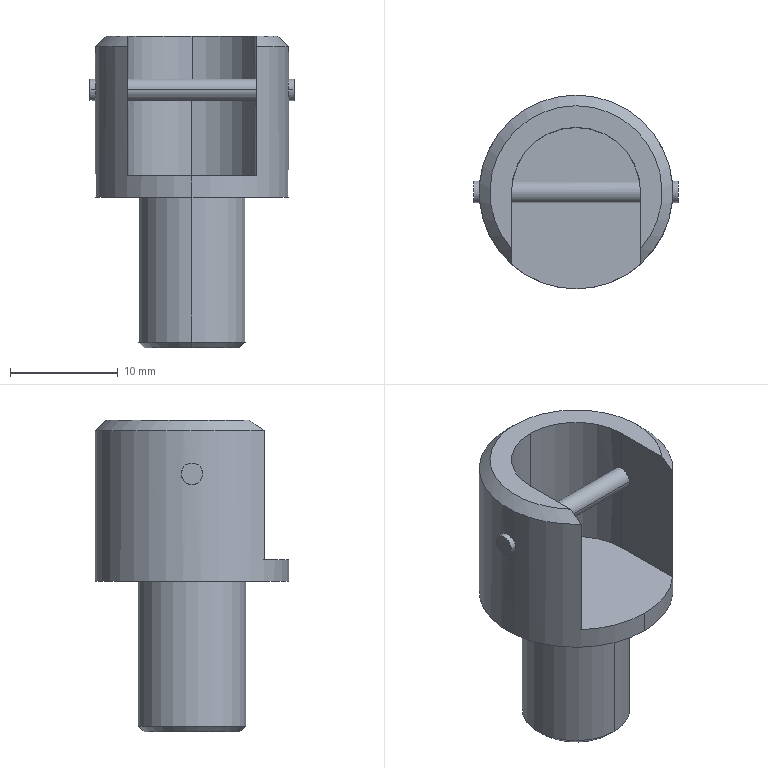Component | SolidWorks | ControlAssembly-1_UWAFN120-1_1_1-1 | 1 solid | 26 faces | box 19 x 18 x 29 mm | volume 2693 mm3 | cylinder 14 | plane 9 | cone 3 | commonest cylinder face diameters 2 x6 5.2 x2 18 x2 10 x2 12 x2
STEP:
#1=CARTESIAN_POINT('',(24.624,0.9121,20.53));
#2=VERTEX_POINT('',#1);
#3=CARTESIAN_POINT('',(24.624,0.7073,20.53));
#4=VERTEX_POINT('',#3);
#5=CARTESIAN_POINT('',(24.624,0.8097,20.53));
#6=DIRECTION('',(-0.00009864,0.,-1.));
#7=DIRECTION('',(0.,-1.,0.));
#8=AXIS2_PLACEMENT_3D('',#5,#6,#7);
#9=CIRCLE('',#8,0.1024);
#10=EDGE_CURVE('',#2,#4,#9,.T.);
#11=ORIENTED_EDGE('',*,*,#10,.F.);
#12=CARTESIAN_POINT('',(24.624,0.9121,20.136));
#13=VERTEX_POINT('',#12);
#14=CARTESIAN_POINT('',(24.624,0.9121,20.53));
#15=DIRECTION('',(-0.00009864,0.,-1.));
#16=VECTOR('',#15,39.37);
#17=LINE('',#14,#16);
#18=EDGE_CURVE('',#2,#13,#17,.T.);
#19=ORIENTED_EDGE('',*,*,#18,.T.);
#20=CARTESIAN_POINT('',(24.624,0.7073,20.136));
#21=VERTEX_POINT('',#20);
#22=CARTESIAN_POINT('',(24.624,0.8097,20.136));
#23=DIRECTION('',(-0.00009864,0.,-1.));
#24=DIRECTION('',(0.,-1.,0.));
#25=AXIS2_PLACEMENT_3D('',#22,#23,#24);
#26=CIRCLE('',#25,0.1024);
#27=EDGE_CURVE('',#13,#21,#26,.T.);
#28=ORIENTED_EDGE('',*,*,#27,.T.);
#29=CARTESIAN_POINT('',(24.624,0.7073,20.53));
#30=DIRECTION('',(-0.00009864,0.,-1.));
#31=VECTOR('',#30,39.37);
#32=LINE('',#29,#31);
#33=EDGE_CURVE('',#4,#21,#32,.T.);
#34=ORIENTED_EDGE('',*,*,#33,.F.);
#35=EDGE_LOOP('',(#11,#19,#28,#34));
#36=FACE_OUTER_BOUND('',#35,.T.);
#37=CARTESIAN_POINT('',(24.624,0.8097,20.53));
#38=DIRECTION('',(-0.00009864,0.,-1.));
#39=DIRECTION('',(0.,-1.,0.));
#40=AXIS2_PLACEMENT_3D('',#37,#38,#39);
#41=CYLINDRICAL_SURFACE('',#40,0.1024);
#42=ADVANCED_FACE('',(#36),#41,.F.);
#43=CARTESIAN_POINT('',(24.272,0.7703,21.081));
#44=VERTEX_POINT('',#43);
#45=CARTESIAN_POINT('',(24.272,0.8491,21.081));
#46=VERTEX_POINT('',#45);
#47=CARTESIAN_POINT('',(24.272,0.7703,21.081));
#48=CARTESIAN_POINT('',(24.272,0.7703,21.076));
#49=CARTESIAN_POINT('',(24.272,0.7714,21.07));
#50=CARTESIAN_POINT('',(24.272,0.7753,21.061));
#51=CARTESIAN_POINT('',(24.271,0.7782,21.057));
#52=CARTESIAN_POINT('',(24.271,0.7855,21.049));
#53=CARTESIAN_POINT('',(24.271,0.7899,21.046));
#54=CARTESIAN_POINT('',(24.27,0.7994,21.042));
#55=CARTESIAN_POINT('',(24.27,0.8045,21.041));
#56=CARTESIAN_POINT('',(24.27,0.8149,21.041));
#57=CARTESIAN_POINT('',(24.27,0.82,21.042));
#58=CARTESIAN_POINT('',(24.271,0.8295,21.046));
#59=CARTESIAN_POINT('',(24.271,0.8339,21.049));
#60=CARTESIAN_POINT('',(24.272,0.8448,21.06));
#61=CARTESIAN_POINT('',(24.272,0.8491,21.07));
#62=CARTESIAN_POINT('',(24.272,0.8491,21.081));
#63=B_SPLINE_CURVE_WITH_KNOTS('',3,(#47,#48,#49,#50,#51,#52,#53,#54,#55,#56,#57,#58,#59,#60,#61,#62),.UNSPECIFIED.,.F.,.F.,(4,2,2,2,2,2,2,4),(0.004692,0.005082,0.005473,0.005864,0.006255,0.006646,0.007037,0.007818),.UNSPECIFIED.);
#64=EDGE_CURVE('',#44,#46,#63,.T.);
#65=ORIENTED_EDGE('',*,*,#64,.T.);
#66=CARTESIAN_POINT('',(24.272,0.8491,21.081));
#67=CARTESIAN_POINT('',(24.272,0.8491,21.086));
#68=CARTESIAN_POINT('',(24.272,0.848,21.091));
#69=CARTESIAN_POINT('',(24.272,0.8441,21.101));
#70=CARTESIAN_POINT('',(24.271,0.8412,21.105));
#71=CARTESIAN_POINT('',(24.271,0.8303,21.116));
#72=CARTESIAN_POINT('',(24.27,0.8201,21.12));
#73=CARTESIAN_POINT('',(24.27,0.8045,21.12));
#74=CARTESIAN_POINT('',(24.27,0.7994,21.119));
#75=CARTESIAN_POINT('',(24.271,0.7898,21.115));
#76=CARTESIAN_POINT('',(24.271,0.7855,21.112));
#77=CARTESIAN_POINT('',(24.271,0.7782,21.105));
#78=CARTESIAN_POINT('',(24.272,0.7753,21.101));
#79=CARTESIAN_POINT('',(24.272,0.7714,21.091));
#80=CARTESIAN_POINT('',(24.272,0.7703,21.086));
#81=CARTESIAN_POINT('',(24.272,0.7703,21.081));
#82=B_SPLINE_CURVE_WITH_KNOTS('',3,(#66,#67,#68,#69,#70,#71,#72,#73,#74,#75,#76,#77,#78,#79,#80,#81),.UNSPECIFIED.,.F.,.F.,(4,2,2,2,2,2,2,4),(0.001563,0.001954,0.002345,0.003127,0.003518,0.00391,0.004301,0.004692),.UNSPECIFIED.);
#83=EDGE_CURVE('',#46,#44,#82,.T.);
#84=ORIENTED_EDGE('',*,*,#83,.T.);
#85=EDGE_LOOP('',(#65,#84));
#86=FACE_BOUND('',#85,.T.);
#87=CARTESIAN_POINT('',(24.388,0.5456,21.238));
#88=VERTEX_POINT('',#87);
#89=CARTESIAN_POINT('',(24.624,1.164,21.238));
#90=VERTEX_POINT('',#89);
#91=CARTESIAN_POINT('',(24.624,0.8097,21.238));
#92=DIRECTION('',(-0.00009864,0.,-1.));
#93=DIRECTION('',(0.,-1.,0.));
#94=AXIS2_PLACEMENT_3D('',#91,#92,#93);
#95=CIRCLE('',#94,0.3543);
#96=EDGE_CURVE('',#88,#90,#95,.T.);
#97=ORIENTED_EDGE('',*,*,#96,.T.);
#98=CARTESIAN_POINT('',(24.624,1.164,20.687));
#99=VERTEX_POINT('',#98);
#100=CARTESIAN_POINT('',(24.624,1.164,20.963));
#101=DIRECTION('',(-0.00009864,0.,-1.));
#102=VECTOR('',#101,39.37);
#103=LINE('',#100,#102);
#104=EDGE_CURVE('',#90,#99,#103,.T.);
#105=ORIENTED_EDGE('',*,*,#104,.T.);
#106=CARTESIAN_POINT('',(24.624,0.4554,20.687));
#107=VERTEX_POINT('',#106);
#108=CARTESIAN_POINT('',(24.624,0.8097,20.687));
#109=DIRECTION('',(0.00009864,-0.,1.));
#110=DIRECTION('',(0.,-1.,0.));
#111=AXIS2_PLACEMENT_3D('',#108,#109,#110);
#112=CIRCLE('',#111,0.3543);
#113=EDGE_CURVE('',#99,#107,#112,.T.);
#114=ORIENTED_EDGE('',*,*,#113,.T.);
#115=CARTESIAN_POINT('',(24.624,0.4554,20.766));
#116=VERTEX_POINT('',#115);
#117=CARTESIAN_POINT('',(24.624,0.4554,20.963));
#118=DIRECTION('',(-0.00009864,0.,-1.));
#119=VECTOR('',#118,39.37);
#120=LINE('',#117,#119);
#121=EDGE_CURVE('',#116,#107,#120,.T.);
#122=ORIENTED_EDGE('',*,*,#121,.F.);
#123=CARTESIAN_POINT('',(24.388,0.5456,20.766));
#124=VERTEX_POINT('',#123);
#125=CARTESIAN_POINT('',(24.624,0.8097,20.766));
#126=DIRECTION('',(-0.00009864,0.,-1.));
#127=DIRECTION('',(0.,-1.,0.));
#128=AXIS2_PLACEMENT_3D('',#125,#126,#127);
#129=CIRCLE('',#128,0.3543);
#130=EDGE_CURVE('',#116,#124,#129,.T.);
#131=ORIENTED_EDGE('',*,*,#130,.T.);
#132=CARTESIAN_POINT('',(24.388,0.5456,20.963));
#133=DIRECTION('',(0.00009864,-0.,1.));
#134=VECTOR('',#133,39.37);
#135=LINE('',#132,#134);
#136=EDGE_CURVE('',#124,#88,#135,.T.);
#137=ORIENTED_EDGE('',*,*,#136,.T.);
#138=EDGE_LOOP('',(#97,#105,#114,#122,#131,#137));
#139=FACE_OUTER_BOUND('',#138,.T.);
#140=CARTESIAN_POINT('',(24.624,0.8097,20.963));
#141=DIRECTION('',(-0.00009864,0.,-1.));
#142=DIRECTION('',(0.,-1.,0.));
#143=AXIS2_PLACEMENT_3D('',#140,#141,#142);
#144=CYLINDRICAL_SURFACE('',#143,0.3543);
#145=ADVANCED_FACE('',(#86,#139),#144,.T.);
#146=CARTESIAN_POINT('',(24.998,0.7703,21.081));
#147=VERTEX_POINT('',#146);
#148=CARTESIAN_POINT('',(24.998,0.8491,21.081));
#149=VERTEX_POINT('',#148);
#150=CARTESIAN_POINT('',(24.998,0.8097,21.081));
#151=DIRECTION('',(-1.,-0.,0.00009864));
#152=DIRECTION('',(0.,-1.,0.));
#153=AXIS2_PLACEMENT_3D('',#150,#151,#152);
#154=CIRCLE('',#153,0.03937);
#155=EDGE_CURVE('',#147,#149,#154,.T.);
#156=ORIENTED_EDGE('',*,*,#155,.T.);
#157=CARTESIAN_POINT('',(24.976,0.8491,21.081));
#158=VERTEX_POINT('',#157);
#159=CARTESIAN_POINT('',(24.624,0.8491,21.081));
#160=DIRECTION('',(-1.,-0.,0.00009864));
#161=VECTOR('',#160,39.37);
#162=LINE('',#159,#161);
#163=EDGE_CURVE('',#149,#158,#162,.T.);
#164=ORIENTED_EDGE('',*,*,#163,.T.);
#165=CARTESIAN_POINT('',(24.976,0.7703,21.081));
#166=VERTEX_POINT('',#165);
#167=CARTESIAN_POINT('',(24.976,0.7703,21.081));
#168=CARTESIAN_POINT('',(24.976,0.7703,21.086));
#169=CARTESIAN_POINT('',(24.977,0.7714,21.091));
#170=CARTESIAN_POINT('',(24.977,0.7753,21.1));
#171=CARTESIAN_POINT('',(24.977,0.7782,21.105));
#172=CARTESIAN_POINT('',(24.978,0.7855,21.112));
#173=CARTESIAN_POINT('',(24.978,0.7899,21.115));
#174=CARTESIAN_POINT('',(24.979,0.7994,21.119));
#175=CARTESIAN_POINT('',(24.979,0.8045,21.12));
#176=CARTESIAN_POINT('',(24.979,0.8149,21.12));
#177=CARTESIAN_POINT('',(24.979,0.82,21.119));
#178=CARTESIAN_POINT('',(24.978,0.8295,21.115));
#179=CARTESIAN_POINT('',(24.978,0.8339,21.112));
#180=CARTESIAN_POINT('',(24.977,0.8448,21.101));
#181=CARTESIAN_POINT('',(24.976,0.8491,21.091));
#182=CARTESIAN_POINT('',(24.976,0.8491,21.081));
#183=B_SPLINE_CURVE_WITH_KNOTS('',3,(#167,#168,#169,#170,#171,#172,#173,#174,#175,#176,#177,#178,#179,#180,#181,#182),.UNSPECIFIED.,.F.,.F.,(4,2,2,2,2,2,2,4),(0.004692,0.005082,0.005473,0.005864,0.006255,0.006646,0.007037,0.007818),.UNSPECIFIED.);
#184=EDGE_CURVE('',#166,#158,#183,.T.);
#185=ORIENTED_EDGE('',*,*,#184,.F.);
#186=CARTESIAN_POINT('',(24.624,0.7703,21.081));
#187=DIRECTION('',(-1.,-0.,0.00009864));
#188=VECTOR('',#187,39.37);
#189=LINE('',#186,#188);
#190=EDGE_CURVE('',#147,#166,#189,.T.);
#191=ORIENTED_EDGE('',*,*,#190,.F.);
#192=EDGE_LOOP('',(#156,#164,#185,#191));
#193=FACE_OUTER_BOUND('',#192,.T.);
#194=CARTESIAN_POINT('',(24.624,0.8097,21.081));
#195=DIRECTION('',(-1.,-0.,0.00009864));
#196=DIRECTION('',(0.,-1.,0.));
#197=AXIS2_PLACEMENT_3D('',#194,#195,#196);
#198=CYLINDRICAL_SURFACE('',#197,0.03937);
#199=ADVANCED_FACE('',(#193),#198,.T.);
#200=ORIENTED_EDGE('',*,*,#83,.F.);
#201=CARTESIAN_POINT('',(24.25,0.8491,21.081));
#202=VERTEX_POINT('',#201);
#203=CARTESIAN_POINT('',(24.624,0.8491,21.081));
#204=DIRECTION('',(-1.,-0.,0.00009864));
#205=VECTOR('',#204,39.37);
#206=LINE('',#203,#205);
#207=EDGE_CURVE('',#46,#202,#206,.T.);
#208=ORIENTED_EDGE('',*,*,#207,.T.);
#209=CARTESIAN_POINT('',(24.25,0.7703,21.081));
#210=VERTEX_POINT('',#209);
#211=CARTESIAN_POINT('',(24.25,0.8097,21.081));
#212=DIRECTION('',(1.,0.,-0.00009864));
#213=DIRECTION('',(0.,-1.,-0.));
#214=AXIS2_PLACEMENT_3D('',#211,#212,#213);
#215=CIRCLE('',#214,0.03937);
#216=EDGE_CURVE('',#202,#210,#215,.T.);
#217=ORIENTED_EDGE('',*,*,#216,.T.);
#218=CARTESIAN_POINT('',(24.624,0.7703,21.081));
#219=DIRECTION('',(-1.,-0.,0.00009864));
#220=VECTOR('',#219,39.37);
#221=LINE('',#218,#220);
#222=EDGE_CURVE('',#44,#210,#221,.T.);
#223=ORIENTED_EDGE('',*,*,#222,.F.);
#224=EDGE_LOOP('',(#200,#208,#217,#223));
#225=FACE_OUTER_BOUND('',#224,.T.);
#226=CARTESIAN_POINT('',(24.624,0.8097,21.081));
#227=DIRECTION('',(-1.,-0.,0.00009864));
#228=DIRECTION('',(0.,-1.,0.));
#229=AXIS2_PLACEMENT_3D('',#226,#227,#228);
#230=CYLINDRICAL_SURFACE('',#229,0.03937);
#231=ADVANCED_FACE('',(#225),#230,.T.);
#232=CARTESIAN_POINT('',(24.624,1.007,20.687));
#233=VERTEX_POINT('',#232);
#234=CARTESIAN_POINT('',(24.624,0.6129,20.687));
#235=VERTEX_POINT('',#234);
#236=CARTESIAN_POINT('',(24.624,0.8097,20.687));
#237=DIRECTION('',(0.00009864,-0.,1.));
#238=DIRECTION('',(0.,-1.,0.));
#239=AXIS2_PLACEMENT_3D('',#236,#237,#238);
#240=CIRCLE('',#239,0.1969);
#241=EDGE_CURVE('',#233,#235,#240,.T.);
#242=ORIENTED_EDGE('',*,*,#241,.F.);
#243=CARTESIAN_POINT('',(24.624,1.007,20.157));
#244=VERTEX_POINT('',#243);
#245=CARTESIAN_POINT('',(24.624,1.007,20.422));
#246=DIRECTION('',(-0.00009864,0.,-1.));
#247=VECTOR('',#246,39.37);
#248=LINE('',#245,#247);
#249=EDGE_CURVE('',#233,#244,#248,.T.);
#250=ORIENTED_EDGE('',*,*,#249,.T.);
#251=CARTESIAN_POINT('',(24.624,0.6129,20.157));
#252=VERTEX_POINT('',#251);
#253=CARTESIAN_POINT('',(24.624,0.8097,20.157));
#254=DIRECTION('',(0.00009864,-0.,1.));
#255=DIRECTION('',(0.,-1.,0.));
#256=AXIS2_PLACEMENT_3D('',#253,#254,#255);
#257=CIRCLE('',#256,0.1969);
#258=EDGE_CURVE('',#244,#252,#257,.T.);
#259=ORIENTED_EDGE('',*,*,#258,.T.);
#260=CARTESIAN_POINT('',(24.624,0.6129,20.422));
#261=DIRECTION('',(-0.00009864,0.,-1.));
#262=VECTOR('',#261,39.37);
#263=LINE('',#260,#262);
#264=EDGE_CURVE('',#235,#252,#263,.T.);
#265=ORIENTED_EDGE('',*,*,#264,.F.);
#266=EDGE_LOOP('',(#242,#250,#259,#265));
#267=FACE_OUTER_BOUND('',#266,.T.);
#268=CARTESIAN_POINT('',(24.624,0.8097,20.422));
#269=DIRECTION('',(-0.00009864,0.,-1.));
#270=DIRECTION('',(0.,-1.,0.));
#271=AXIS2_PLACEMENT_3D('',#268,#269,#270);
#272=CYLINDRICAL_SURFACE('',#271,0.1969);
#273=ADVANCED_FACE('',(#267),#272,.T.);
#274=CARTESIAN_POINT('',(24.624,0.9852,20.136));
#275=VERTEX_POINT('',#274);
#276=CARTESIAN_POINT('',(24.624,0.6342,20.136));
#277=VERTEX_POINT('',#276);
#278=CARTESIAN_POINT('',(24.624,0.8097,20.136));
#279=DIRECTION('',(0.00009864,0.,1.));
#280=DIRECTION('',(0.,1.,0.));
#281=AXIS2_PLACEMENT_3D('',#278,#279,#280);
#282=CIRCLE('',#281,0.1755);
#283=EDGE_CURVE('',#275,#277,#282,.T.);
#284=ORIENTED_EDGE('',*,*,#283,.T.);
#285=CARTESIAN_POINT('',(24.624,0.6129,20.157));
#286=DIRECTION('',(0.00006975,-0.7071,0.7071));
#287=VECTOR('',#286,39.37);
#288=LINE('',#285,#287);
#289=EDGE_CURVE('',#277,#252,#288,.T.);
#290=ORIENTED_EDGE('',*,*,#289,.T.);
#291=ORIENTED_EDGE('',*,*,#258,.F.);
#292=CARTESIAN_POINT('',(24.624,1.007,20.157));
#293=DIRECTION('',(0.00006975,0.7071,0.7071));
#294=VECTOR('',#293,39.37);
#295=LINE('',#292,#294);
#296=EDGE_CURVE('',#275,#244,#295,.T.);
#297=ORIENTED_EDGE('',*,*,#296,.F.);
#298=EDGE_LOOP('',(#284,#290,#291,#297));
#299=FACE_OUTER_BOUND('',#298,.T.);
#300=CARTESIAN_POINT('',(24.624,0.8097,20.157));
#301=DIRECTION('',(0.00009864,0.,1.));
#302=DIRECTION('',(0.,1.,0.));
#303=AXIS2_PLACEMENT_3D('',#300,#301,#302);
#304=CONICAL_SURFACE('',#303,0.1969,0.7854);
#305=ADVANCED_FACE('',(#299),#304,.T.);
#306=CARTESIAN_POINT('',(24.861,0.8097,21.12));
#307=VERTEX_POINT('',#306);
#308=CARTESIAN_POINT('',(24.857,0.8491,21.081));
#309=VERTEX_POINT('',#308);
#310=CARTESIAN_POINT('',(24.861,0.8097,21.12));
#311=CARTESIAN_POINT('',(24.861,0.8149,21.12));
#312=CARTESIAN_POINT('',(24.86,0.82,21.119));
#313=CARTESIAN_POINT('',(24.86,0.8296,21.115));
#314=CARTESIAN_POINT('',(24.859,0.8339,21.112));
#315=CARTESIAN_POINT('',(24.858,0.8412,21.105));
#316=CARTESIAN_POINT('',(24.858,0.8441,21.1));
#317=CARTESIAN_POINT('',(24.857,0.848,21.091));
#318=CARTESIAN_POINT('',(24.857,0.8491,21.086));
#319=CARTESIAN_POINT('',(24.857,0.8491,21.081));
#320=B_SPLINE_CURVE_WITH_KNOTS('',3,(#310,#311,#312,#313,#314,#315,#316,#317,#318,#319),.UNSPECIFIED.,.F.,.F.,(4,2,2,2,4),(0.,0.0003916,0.0007832,0.001175,0.001566),.UNSPECIFIED.);
#321=EDGE_CURVE('',#307,#309,#320,.T.);
#322=ORIENTED_EDGE('',*,*,#321,.T.);
#323=CARTESIAN_POINT('',(24.391,0.8491,21.081));
#324=VERTEX_POINT('',#323);
#325=CARTESIAN_POINT('',(24.624,0.8491,21.081));
#326=DIRECTION('',(-1.,-0.,0.00009864));
#327=VECTOR('',#326,39.37);
#328=LINE('',#325,#327);
#329=EDGE_CURVE('',#309,#324,#328,.T.);
#330=ORIENTED_EDGE('',*,*,#329,.T.);
#331=CARTESIAN_POINT('',(24.388,0.8097,21.12));
#332=VERTEX_POINT('',#331);
#333=CARTESIAN_POINT('',(24.391,0.8491,21.081));
#334=CARTESIAN_POINT('',(24.391,0.8491,21.086));
#335=CARTESIAN_POINT('',(24.391,0.848,21.091));
#336=CARTESIAN_POINT('',(24.391,0.8441,21.101));
#337=CARTESIAN_POINT('',(24.39,0.8412,21.105));
#338=CARTESIAN_POINT('',(24.389,0.8339,21.112));
#339=CARTESIAN_POINT('',(24.389,0.8296,21.115));
#340=CARTESIAN_POINT('',(24.388,0.82,21.119));
#341=CARTESIAN_POINT('',(24.388,0.8149,21.12));
#342=CARTESIAN_POINT('',(24.388,0.8097,21.12));
#343=B_SPLINE_CURVE_WITH_KNOTS('',3,(#333,#334,#335,#336,#337,#338,#339,#340,#341,#342),.UNSPECIFIED.,.F.,.F.,(4,2,2,2,4),(0.001566,0.001958,0.002349,0.00274,0.003131),.UNSPECIFIED.);
#344=EDGE_CURVE('',#324,#332,#343,.T.);
#345=ORIENTED_EDGE('',*,*,#344,.T.);
#346=CARTESIAN_POINT('',(24.388,0.7703,21.081));
#347=VERTEX_POINT('',#346);
#348=CARTESIAN_POINT('',(24.388,0.8097,21.081));
#349=DIRECTION('',(1.,0.,-0.00009864));
#350=DIRECTION('',(0.,-1.,-0.));
#351=AXIS2_PLACEMENT_3D('',#348,#349,#350);
#352=CIRCLE('',#351,0.03937);
#353=EDGE_CURVE('',#332,#347,#352,.T.);
#354=ORIENTED_EDGE('',*,*,#353,.T.);
#355=CARTESIAN_POINT('',(24.861,0.7703,21.081));
#356=VERTEX_POINT('',#355);
#357=CARTESIAN_POINT('',(24.624,0.7703,21.081));
#358=DIRECTION('',(-1.,-0.,0.00009864));
#359=VECTOR('',#358,39.37);
#360=LINE('',#357,#359);
#361=EDGE_CURVE('',#356,#347,#360,.T.);
#362=ORIENTED_EDGE('',*,*,#361,.F.);
#363=CARTESIAN_POINT('',(24.861,0.8097,21.081));
#364=DIRECTION('',(-1.,-0.,0.00009864));
#365=DIRECTION('',(0.,-1.,0.));
#366=AXIS2_PLACEMENT_3D('',#363,#364,#365);
#367=CIRCLE('',#366,0.03937);
#368=EDGE_CURVE('',#356,#307,#367,.T.);
#369=ORIENTED_EDGE('',*,*,#368,.T.);
#370=EDGE_LOOP('',(#322,#330,#345,#354,#362,#369));
#371=FACE_OUTER_BOUND('',#370,.T.);
#372=CARTESIAN_POINT('',(24.624,0.8097,21.081));
#373=DIRECTION('',(-1.,-0.,0.00009864));
#374=DIRECTION('',(0.,-1.,0.));
#375=AXIS2_PLACEMENT_3D('',#372,#373,#374);
#376=CYLINDRICAL_SURFACE('',#375,0.03937);
#377=ADVANCED_FACE('',(#371),#376,.T.);
#378=CARTESIAN_POINT('',(24.624,1.046,20.766));
#379=VERTEX_POINT('',#378);
#380=CARTESIAN_POINT('',(24.388,0.8097,20.766));
#381=VERTEX_POINT('',#380);
#382=CARTESIAN_POINT('',(24.624,0.8097,20.766));
#383=DIRECTION('',(0.00009864,-0.,1.));
#384=DIRECTION('',(0.,1.,0.));
#385=AXIS2_PLACEMENT_3D('',#382,#383,#384);
#386=CIRCLE('',#385,0.2362);
#387=EDGE_CURVE('',#379,#381,#386,.T.);
#388=ORIENTED_EDGE('',*,*,#387,.F.);
#389=CARTESIAN_POINT('',(24.624,1.046,21.278));
#390=VERTEX_POINT('',#389);
#391=CARTESIAN_POINT('',(24.624,1.046,21.278));
#392=DIRECTION('',(0.00009864,-0.,1.));
#393=VECTOR('',#392,39.37);
#394=LINE('',#391,#393);
#395=EDGE_CURVE('',#379,#390,#394,.T.);
#396=ORIENTED_EDGE('',*,*,#395,.T.);
#397=CARTESIAN_POINT('',(24.388,0.8097,21.278));
#398=VERTEX_POINT('',#397);
#399=CARTESIAN_POINT('',(24.624,0.8097,21.278));
#400=DIRECTION('',(-0.00009864,0.,-1.));
#401=DIRECTION('',(0.,1.,0.));
#402=AXIS2_PLACEMENT_3D('',#399,#400,#401);
#403=CIRCLE('',#402,0.2362);
#404=EDGE_CURVE('',#398,#390,#403,.T.);
#405=ORIENTED_EDGE('',*,*,#404,.F.);
#406=CARTESIAN_POINT('',(24.388,0.8097,21.278));
#407=DIRECTION('',(-0.00009864,0.,-1.));
#408=VECTOR('',#407,39.37);
#409=LINE('',#406,#408);
#410=EDGE_CURVE('',#398,#332,#409,.T.);
#411=ORIENTED_EDGE('',*,*,#410,.T.);
#412=ORIENTED_EDGE('',*,*,#344,.F.);
#413=CARTESIAN_POINT('',(24.388,0.8097,21.041));
#414=VERTEX_POINT('',#413);
#415=CARTESIAN_POINT('',(24.388,0.8097,21.041));
#416=CARTESIAN_POINT('',(24.388,0.8149,21.041));
#417=CARTESIAN_POINT('',(24.388,0.82,21.042));
#418=CARTESIAN_POINT('',(24.389,0.8296,21.046));
#419=CARTESIAN_POINT('',(24.389,0.8339,21.049));
#420=CARTESIAN_POINT('',(24.39,0.8412,21.057));
#421=CARTESIAN_POINT('',(24.391,0.8441,21.061));
#422=CARTESIAN_POINT('',(24.391,0.848,21.07));
#423=CARTESIAN_POINT('',(24.391,0.8491,21.076));
#424=CARTESIAN_POINT('',(24.391,0.8491,21.081));
#425=B_SPLINE_CURVE_WITH_KNOTS('',3,(#415,#416,#417,#418,#419,#420,#421,#422,#423,#424),.UNSPECIFIED.,.F.,.F.,(4,2,2,2,4),(0.,0.0003916,0.0007832,0.001175,0.001566),.UNSPECIFIED.);
#426=EDGE_CURVE('',#414,#324,#425,.T.);
#427=ORIENTED_EDGE('',*,*,#426,.F.);
#428=CARTESIAN_POINT('',(24.388,0.8097,21.278));
#429=DIRECTION('',(-0.00009864,0.,-1.));
#430=VECTOR('',#429,39.37);
#431=LINE('',#428,#430);
#432=EDGE_CURVE('',#414,#381,#431,.T.);
#433=ORIENTED_EDGE('',*,*,#432,.T.);
#434=EDGE_LOOP('',(#388,#396,#405,#411,#412,#427,#433));
#435=FACE_OUTER_BOUND('',#434,.T.);
#436=CARTESIAN_POINT('',(24.624,0.8097,21.278));
#437=DIRECTION('',(0.00009864,-0.,1.));
#438=DIRECTION('',(0.,1.,0.));
#439=AXIS2_PLACEMENT_3D('',#436,#437,#438);
#440=CYLINDRICAL_SURFACE('',#439,0.2362);
#441=ADVANCED_FACE('',(#435),#440,.F.);
#442=ORIENTED_EDGE('',*,*,#104,.F.);
#443=CARTESIAN_POINT('',(24.861,0.5456,21.238));
#444=VERTEX_POINT('',#443);
#445=CARTESIAN_POINT('',(24.624,0.8097,21.238));
#446=DIRECTION('',(-0.00009864,0.,-1.));
#447=DIRECTION('',(0.,-1.,0.));
#448=AXIS2_PLACEMENT_3D('',#445,#446,#447);
#449=CIRCLE('',#448,0.3543);
#450=EDGE_CURVE('',#90,#444,#449,.T.);
#451=ORIENTED_EDGE('',*,*,#450,.T.);
#452=CARTESIAN_POINT('',(24.861,0.5456,20.766));
#453=VERTEX_POINT('',#452);
#454=CARTESIAN_POINT('',(24.861,0.5456,20.963));
#455=DIRECTION('',(-0.00009864,0.,-1.));
#456=VECTOR('',#455,39.37);
#457=LINE('',#454,#456);
#458=EDGE_CURVE('',#444,#453,#457,.T.);
#459=ORIENTED_EDGE('',*,*,#458,.T.);
#460=CARTESIAN_POINT('',(24.624,0.8097,20.766));
#461=DIRECTION('',(-0.00009864,0.,-1.));
#462=DIRECTION('',(0.,-1.,0.));
#463=AXIS2_PLACEMENT_3D('',#460,#461,#462);
#464=CIRCLE('',#463,0.3543);
#465=EDGE_CURVE('',#453,#116,#464,.T.);
#466=ORIENTED_EDGE('',*,*,#465,.T.);
#467=ORIENTED_EDGE('',*,*,#121,.T.);
#468=CARTESIAN_POINT('',(24.624,0.8097,20.687));
#469=DIRECTION('',(0.00009864,-0.,1.));
#470=DIRECTION('',(0.,-1.,0.));
#471=AXIS2_PLACEMENT_3D('',#468,#469,#470);
#472=CIRCLE('',#471,0.3543);
#473=EDGE_CURVE('',#107,#99,#472,.T.);
#474=ORIENTED_EDGE('',*,*,#473,.T.);
#475=EDGE_LOOP('',(#442,#451,#459,#466,#467,#474));
#476=FACE_OUTER_BOUND('',#475,.T.);
#477=ORIENTED_EDGE('',*,*,#184,.T.);
#478=CARTESIAN_POINT('',(24.976,0.8491,21.081));
#479=CARTESIAN_POINT('',(24.976,0.8491,21.075));
#480=CARTESIAN_POINT('',(24.977,0.848,21.07));
#481=CARTESIAN_POINT('',(24.977,0.8441,21.061));
#482=CARTESIAN_POINT('',(24.977,0.8412,21.056));
#483=CARTESIAN_POINT('',(24.978,0.8303,21.046));
#484=CARTESIAN_POINT('',(24.979,0.8201,21.041));
#485=CARTESIAN_POINT('',(24.979,0.8045,21.041));
#486=CARTESIAN_POINT('',(24.979,0.7994,21.042));
#487=CARTESIAN_POINT('',(24.978,0.7898,21.046));
#488=CARTESIAN_POINT('',(24.978,0.7855,21.049));
#489=CARTESIAN_POINT('',(24.977,0.7782,21.056));
#490=CARTESIAN_POINT('',(24.977,0.7753,21.061));
#491=CARTESIAN_POINT('',(24.977,0.7714,21.07));
#492=CARTESIAN_POINT('',(24.976,0.7703,21.076));
#493=CARTESIAN_POINT('',(24.976,0.7703,21.081));
#494=B_SPLINE_CURVE_WITH_KNOTS('',3,(#478,#479,#480,#481,#482,#483,#484,#485,#486,#487,#488,#489,#490,#491,#492,#493),.UNSPECIFIED.,.F.,.F.,(4,2,2,2,2,2,2,4),(0.001563,0.001954,0.002345,0.003127,0.003518,0.00391,0.004301,0.004692),.UNSPECIFIED.);
#495=EDGE_CURVE('',#158,#166,#494,.T.);
#496=ORIENTED_EDGE('',*,*,#495,.T.);
#497=EDGE_LOOP('',(#477,#496));
#498=FACE_BOUND('',#497,.T.);
#499=CARTESIAN_POINT('',(24.624,0.8097,20.963));
#500=DIRECTION('',(-0.00009864,0.,-1.));
#501=DIRECTION('',(0.,-1.,0.));
#502=AXIS2_PLACEMENT_3D('',#499,#500,#501);
#503=CYLINDRICAL_SURFACE('',#502,0.3543);
#504=ADVANCED_FACE('',(#476,#498),#503,.T.);
#505=ORIENTED_EDGE('',*,*,#473,.F.);
#506=ORIENTED_EDGE('',*,*,#113,.F.);
#507=EDGE_LOOP('',(#505,#506));
#508=FACE_OUTER_BOUND('',#507,.T.);
#509=CARTESIAN_POINT('',(24.624,0.8097,20.687));
#510=DIRECTION('',(0.00009864,-0.,1.));
#511=DIRECTION('',(0.,-1.,0.));
#512=AXIS2_PLACEMENT_3D('',#509,#510,#511);
#513=CIRCLE('',#512,0.1969);
#514=EDGE_CURVE('',#235,#233,#513,.T.);
#515=ORIENTED_EDGE('',*,*,#514,.T.);
#516=ORIENTED_EDGE('',*,*,#241,.T.);
#517=EDGE_LOOP('',(#515,#516));
#518=FACE_BOUND('',#517,.T.);
#519=CARTESIAN_POINT('',(24.447,0.8097,20.687));
#520=DIRECTION('',(-0.00009864,0.,-1.));
#521=DIRECTION('',(0.,-1.,-0.));
#522=AXIS2_PLACEMENT_3D('',#519,#520,#521);
#523=PLANE('',#522);
#524=ADVANCED_FACE('',(#508,#518),#523,.T.);
#525=ORIENTED_EDGE('',*,*,#163,.F.);
#526=CARTESIAN_POINT('',(24.998,0.8097,21.081));
#527=DIRECTION('',(-1.,-0.,0.00009864));
#528=DIRECTION('',(0.,-1.,0.));
#529=AXIS2_PLACEMENT_3D('',#526,#527,#528);
#530=CIRCLE('',#529,0.03937);
#531=EDGE_CURVE('',#149,#147,#530,.T.);
#532=ORIENTED_EDGE('',*,*,#531,.T.);
#533=ORIENTED_EDGE('',*,*,#190,.T.);
#534=ORIENTED_EDGE('',*,*,#495,.F.);
#535=EDGE_LOOP('',(#525,#532,#533,#534));
#536=FACE_OUTER_BOUND('',#535,.T.);
#537=CARTESIAN_POINT('',(24.624,0.8097,21.081));
#538=DIRECTION('',(-1.,-0.,0.00009864));
#539=DIRECTION('',(0.,-1.,0.));
#540=AXIS2_PLACEMENT_3D('',#537,#538,#539);
#541=CYLINDRICAL_SURFACE('',#540,0.03937);
#542=ADVANCED_FACE('',(#536),#541,.T.);
#543=CARTESIAN_POINT('',(24.388,0.6014,21.278));
#544=VERTEX_POINT('',#543);
#545=CARTESIAN_POINT('',(24.861,0.6014,21.278));
#546=VERTEX_POINT('',#545);
#547=CARTESIAN_POINT('',(24.624,0.8097,21.278));
#548=DIRECTION('',(-0.00009864,-0.,-1.));
#549=DIRECTION('',(0.,-1.,0.));
#550=AXIS2_PLACEMENT_3D('',#547,#548,#549);
#551=CIRCLE('',#550,0.315);
#552=EDGE_CURVE('',#544,#546,#551,.T.);
#553=ORIENTED_EDGE('',*,*,#552,.T.);
#554=CARTESIAN_POINT('',(24.861,0.6014,21.278));
#555=CARTESIAN_POINT('',(24.861,0.5824,21.265));
#556=CARTESIAN_POINT('',(24.861,0.5639,21.252));
#557=CARTESIAN_POINT('',(24.861,0.5456,21.238));
#558=B_SPLINE_CURVE_WITH_KNOTS('',3,(#554,#555,#556,#557),.UNSPECIFIED.,.F.,.F.,(4,4),(0.,0.001734),.UNSPECIFIED.);
#559=EDGE_CURVE('',#546,#444,#558,.T.);
#560=ORIENTED_EDGE('',*,*,#559,.T.);
#561=ORIENTED_EDGE('',*,*,#450,.F.);
#562=ORIENTED_EDGE('',*,*,#96,.F.);
#563=CARTESIAN_POINT('',(24.388,0.5456,21.238));
#564=CARTESIAN_POINT('',(24.388,0.5639,21.252));
#565=CARTESIAN_POINT('',(24.388,0.5824,21.265));
#566=CARTESIAN_POINT('',(24.388,0.6014,21.278));
#567=B_SPLINE_CURVE_WITH_KNOTS('',3,(#563,#564,#565,#566),.UNSPECIFIED.,.F.,.F.,(4,4),(0.,0.001734),.UNSPECIFIED.);
#568=EDGE_CURVE('',#88,#544,#567,.T.);
#569=ORIENTED_EDGE('',*,*,#568,.T.);
#570=EDGE_LOOP('',(#553,#560,#561,#562,#569));
#571=FACE_OUTER_BOUND('',#570,.T.);
#572=CARTESIAN_POINT('',(24.624,0.8097,21.238));
#573=DIRECTION('',(-0.00009864,-0.,-1.));
#574=DIRECTION('',(0.,-1.,0.));
#575=AXIS2_PLACEMENT_3D('',#572,#573,#574);
#576=CONICAL_SURFACE('',#575,0.3543,0.7854);
#577=ADVANCED_FACE('',(#571),#576,.T.);
#578=ORIENTED_EDGE('',*,*,#207,.F.);
#579=ORIENTED_EDGE('',*,*,#64,.F.);
#580=ORIENTED_EDGE('',*,*,#222,.T.);
#581=CARTESIAN_POINT('',(24.25,0.8097,21.081));
#582=DIRECTION('',(1.,0.,-0.00009864));
#583=DIRECTION('',(0.,-1.,0.));
#584=AXIS2_PLACEMENT_3D('',#581,#582,#583);
#585=CIRCLE('',#584,0.03937);
#586=EDGE_CURVE('',#210,#202,#585,.T.);
#587=ORIENTED_EDGE('',*,*,#586,.T.);
#588=EDGE_LOOP('',(#578,#579,#580,#587));
#589=FACE_OUTER_BOUND('',#588,.T.);
#590=CARTESIAN_POINT('',(24.624,0.8097,21.081));
#591=DIRECTION('',(-1.,-0.,0.00009864));
#592=DIRECTION('',(0.,-1.,0.));
#593=AXIS2_PLACEMENT_3D('',#590,#591,#592);
#594=CYLINDRICAL_SURFACE('',#593,0.03937);
#595=ADVANCED_FACE('',(#589),#594,.T.);
#596=ORIENTED_EDGE('',*,*,#249,.F.);
#597=ORIENTED_EDGE('',*,*,#514,.F.);
#598=ORIENTED_EDGE('',*,*,#264,.T.);
#599=CARTESIAN_POINT('',(24.624,0.8097,20.157));
#600=DIRECTION('',(0.00009864,-0.,1.));
#601=DIRECTION('',(0.,-1.,0.));
#602=AXIS2_PLACEMENT_3D('',#599,#600,#601);
#603=CIRCLE('',#602,0.1969);
#604=EDGE_CURVE('',#252,#244,#603,.T.);
#605=ORIENTED_EDGE('',*,*,#604,.T.);
#606=EDGE_LOOP('',(#596,#597,#598,#605));
#607=FACE_OUTER_BOUND('',#606,.T.);
#608=CARTESIAN_POINT('',(24.624,0.8097,20.422));
#609=DIRECTION('',(-0.00009864,0.,-1.));
#610=DIRECTION('',(0.,-1.,0.));
#611=AXIS2_PLACEMENT_3D('',#608,#609,#610);
#612=CYLINDRICAL_SURFACE('',#611,0.1969);
#613=ADVANCED_FACE('',(#607),#612,.T.);
#614=ORIENTED_EDGE('',*,*,#410,.F.);
#615=CARTESIAN_POINT('',(24.388,0.8097,21.278));
#616=DIRECTION('',(0.,1.,0.));
#617=VECTOR('',#616,39.37);
#618=LINE('',#615,#617);
#619=EDGE_CURVE('',#544,#398,#618,.T.);
#620=ORIENTED_EDGE('',*,*,#619,.F.);
#621=ORIENTED_EDGE('',*,*,#568,.F.);
#622=ORIENTED_EDGE('',*,*,#136,.F.);
#623=CARTESIAN_POINT('',(24.388,0.8097,20.766));
#624=DIRECTION('',(-0.,-1.,-0.));
#625=VECTOR('',#624,39.37);
#626=LINE('',#623,#625);
#627=EDGE_CURVE('',#381,#124,#626,.T.);
#628=ORIENTED_EDGE('',*,*,#627,.F.);
#629=ORIENTED_EDGE('',*,*,#432,.F.);
#630=CARTESIAN_POINT('',(24.388,0.8097,21.081));
#631=DIRECTION('',(1.,0.,-0.00009864));
#632=DIRECTION('',(0.,-1.,0.));
#633=AXIS2_PLACEMENT_3D('',#630,#631,#632);
#634=CIRCLE('',#633,0.03937);
#635=EDGE_CURVE('',#347,#414,#634,.T.);
#636=ORIENTED_EDGE('',*,*,#635,.F.);
#637=ORIENTED_EDGE('',*,*,#353,.F.);
#638=EDGE_LOOP('',(#614,#620,#621,#622,#628,#629,#636,#637));
#639=FACE_OUTER_BOUND('',#638,.T.);
#640=CARTESIAN_POINT('',(24.388,0.8097,21.278));
#641=DIRECTION('',(-1.,0.,0.00009864));
#642=DIRECTION('',(-0.,-1.,-0.));
#643=AXIS2_PLACEMENT_3D('',#640,#641,#642);
#644=PLANE('',#643);
#645=ADVANCED_FACE('',(#639),#644,.F.);
#646=CARTESIAN_POINT('',(24.861,0.8097,20.766));
#647=VERTEX_POINT('',#646);
#648=CARTESIAN_POINT('',(24.624,0.8097,20.766));
#649=DIRECTION('',(0.00009864,-0.,1.));
#650=DIRECTION('',(0.,1.,0.));
#651=AXIS2_PLACEMENT_3D('',#648,#649,#650);
#652=CIRCLE('',#651,0.2362);
#653=EDGE_CURVE('',#647,#379,#652,.T.);
#654=ORIENTED_EDGE('',*,*,#653,.T.);
#655=ORIENTED_EDGE('',*,*,#387,.T.);
#656=ORIENTED_EDGE('',*,*,#627,.T.);
#657=ORIENTED_EDGE('',*,*,#130,.F.);
#658=ORIENTED_EDGE('',*,*,#465,.F.);
#659=CARTESIAN_POINT('',(24.861,0.8097,20.766));
#660=DIRECTION('',(-0.,1.,0.));
#661=VECTOR('',#660,39.37);
#662=LINE('',#659,#661);
#663=EDGE_CURVE('',#453,#647,#662,.T.);
#664=ORIENTED_EDGE('',*,*,#663,.T.);
#665=EDGE_LOOP('',(#654,#655,#656,#657,#658,#664));
#666=FACE_OUTER_BOUND('',#665,.T.);
#667=CARTESIAN_POINT('',(24.624,0.8097,20.766));
#668=DIRECTION('',(0.00009864,-0.,1.));
#669=DIRECTION('',(-0.,1.,0.));
#670=AXIS2_PLACEMENT_3D('',#667,#668,#669);
#671=PLANE('',#670);
#672=ADVANCED_FACE('',(#666),#671,.T.);
#673=CARTESIAN_POINT('',(24.861,0.8097,21.041));
#674=VERTEX_POINT('',#673);
#675=CARTESIAN_POINT('',(24.861,0.8097,21.278));
#676=DIRECTION('',(0.00009864,-0.,1.));
#677=VECTOR('',#676,39.37);
#678=LINE('',#675,#677);
#679=EDGE_CURVE('',#647,#674,#678,.T.);
#680=ORIENTED_EDGE('',*,*,#679,.F.);
#681=ORIENTED_EDGE('',*,*,#663,.F.);
#682=ORIENTED_EDGE('',*,*,#458,.F.);
#683=ORIENTED_EDGE('',*,*,#559,.F.);
#684=CARTESIAN_POINT('',(24.861,0.8097,21.278));
#685=VERTEX_POINT('',#684);
#686=CARTESIAN_POINT('',(24.861,0.4554,21.278));
#687=DIRECTION('',(-0.,-1.,-0.));
#688=VECTOR('',#687,39.37);
#689=LINE('',#686,#688);
#690=EDGE_CURVE('',#685,#546,#689,.T.);
#691=ORIENTED_EDGE('',*,*,#690,.F.);
#692=CARTESIAN_POINT('',(24.861,0.8097,21.278));
#693=DIRECTION('',(0.00009864,-0.,1.));
#694=VECTOR('',#693,39.37);
#695=LINE('',#692,#694);
#696=EDGE_CURVE('',#307,#685,#695,.T.);
#697=ORIENTED_EDGE('',*,*,#696,.F.);
#698=ORIENTED_EDGE('',*,*,#368,.F.);
#699=CARTESIAN_POINT('',(24.861,0.8097,21.081));
#700=DIRECTION('',(-1.,-0.,0.00009864));
#701=DIRECTION('',(0.,-1.,0.));
#702=AXIS2_PLACEMENT_3D('',#699,#700,#701);
#703=CIRCLE('',#702,0.03937);
#704=EDGE_CURVE('',#674,#356,#703,.T.);
#705=ORIENTED_EDGE('',*,*,#704,.F.);
#706=EDGE_LOOP('',(#680,#681,#682,#683,#691,#697,#698,#705));
#707=FACE_OUTER_BOUND('',#706,.T.);
#708=CARTESIAN_POINT('',(24.861,0.4554,21.278));
#709=DIRECTION('',(1.,-0.,-0.00009864));
#710=DIRECTION('',(0.,1.,0.));
#711=AXIS2_PLACEMENT_3D('',#708,#709,#710);
#712=PLANE('',#711);
#713=ADVANCED_FACE('',(#707),#712,.F.);
#714=ORIENTED_EDGE('',*,*,#155,.F.);
#715=ORIENTED_EDGE('',*,*,#531,.F.);
#716=EDGE_LOOP('',(#714,#715));
#717=FACE_OUTER_BOUND('',#716,.T.);
#718=CARTESIAN_POINT('',(24.998,0.8097,21.1));
#719=DIRECTION('',(1.,0.,-0.00009864));
#720=DIRECTION('',(-0.,1.,0.));
#721=AXIS2_PLACEMENT_3D('',#718,#719,#720);
#722=PLANE('',#721);
#723=ADVANCED_FACE('',(#717),#722,.T.);
#724=ORIENTED_EDGE('',*,*,#552,.F.);
#725=ORIENTED_EDGE('',*,*,#619,.T.);
#726=ORIENTED_EDGE('',*,*,#404,.T.);
#727=CARTESIAN_POINT('',(24.624,0.8097,21.278));
#728=DIRECTION('',(-0.00009864,0.,-1.));
#729=DIRECTION('',(0.,1.,0.));
#730=AXIS2_PLACEMENT_3D('',#727,#728,#729);
#731=CIRCLE('',#730,0.2362);
#732=EDGE_CURVE('',#390,#685,#731,.T.);
#733=ORIENTED_EDGE('',*,*,#732,.T.);
#734=ORIENTED_EDGE('',*,*,#690,.T.);
#735=EDGE_LOOP('',(#724,#725,#726,#733,#734));
#736=FACE_OUTER_BOUND('',#735,.T.);
#737=CARTESIAN_POINT('',(24.467,0.8097,21.278));
#738=DIRECTION('',(0.00009864,-0.,1.));
#739=DIRECTION('',(-0.,1.,0.));
#740=AXIS2_PLACEMENT_3D('',#737,#738,#739);
#741=PLANE('',#740);
#742=ADVANCED_FACE('',(#736),#741,.T.);
#743=ORIENTED_EDGE('',*,*,#586,.F.);
#744=ORIENTED_EDGE('',*,*,#216,.F.);
#745=EDGE_LOOP('',(#743,#744));
#746=FACE_OUTER_BOUND('',#745,.T.);
#747=CARTESIAN_POINT('',(24.25,0.8097,21.1));
#748=DIRECTION('',(-1.,-0.,0.00009864));
#749=DIRECTION('',(0.,-1.,-0.));
#750=AXIS2_PLACEMENT_3D('',#747,#748,#749);
#751=PLANE('',#750);
#752=ADVANCED_FACE('',(#746),#751,.T.);
#753=ORIENTED_EDGE('',*,*,#289,.F.);
#754=CARTESIAN_POINT('',(24.624,0.8097,20.136));
#755=DIRECTION('',(0.00009864,0.,1.));
#756=DIRECTION('',(0.,1.,0.));
#757=AXIS2_PLACEMENT_3D('',#754,#755,#756);
#758=CIRCLE('',#757,0.1755);
#759=EDGE_CURVE('',#277,#275,#758,.T.);
#760=ORIENTED_EDGE('',*,*,#759,.T.);
#761=ORIENTED_EDGE('',*,*,#296,.T.);
#762=ORIENTED_EDGE('',*,*,#604,.F.);
#763=EDGE_LOOP('',(#753,#760,#761,#762));
#764=FACE_OUTER_BOUND('',#763,.T.);
#765=CARTESIAN_POINT('',(24.624,0.8097,20.157));
#766=DIRECTION('',(0.00009864,0.,1.));
#767=DIRECTION('',(0.,1.,0.));
#768=AXIS2_PLACEMENT_3D('',#765,#766,#767);
#769=CONICAL_SURFACE('',#768,0.1969,0.7854);
#770=ADVANCED_FACE('',(#764),#769,.T.);
#771=ORIENTED_EDGE('',*,*,#329,.F.);
#772=CARTESIAN_POINT('',(24.857,0.8491,21.081));
#773=CARTESIAN_POINT('',(24.857,0.8491,21.076));
#774=CARTESIAN_POINT('',(24.857,0.848,21.07));
#775=CARTESIAN_POINT('',(24.858,0.8441,21.061));
#776=CARTESIAN_POINT('',(24.858,0.8412,21.057));
#777=CARTESIAN_POINT('',(24.859,0.8339,21.049));
#778=CARTESIAN_POINT('',(24.86,0.8296,21.046));
#779=CARTESIAN_POINT('',(24.86,0.82,21.042));
#780=CARTESIAN_POINT('',(24.861,0.8149,21.041));
#781=CARTESIAN_POINT('',(24.861,0.8097,21.041));
#782=B_SPLINE_CURVE_WITH_KNOTS('',3,(#772,#773,#774,#775,#776,#777,#778,#779,#780,#781),.UNSPECIFIED.,.F.,.F.,(4,2,2,2,4),(0.001566,0.001958,0.002349,0.00274,0.003131),.UNSPECIFIED.);
#783=EDGE_CURVE('',#309,#674,#782,.T.);
#784=ORIENTED_EDGE('',*,*,#783,.T.);
#785=ORIENTED_EDGE('',*,*,#704,.T.);
#786=ORIENTED_EDGE('',*,*,#361,.T.);
#787=ORIENTED_EDGE('',*,*,#635,.T.);
#788=ORIENTED_EDGE('',*,*,#426,.T.);
#789=EDGE_LOOP('',(#771,#784,#785,#786,#787,#788));
#790=FACE_OUTER_BOUND('',#789,.T.);
#791=CARTESIAN_POINT('',(24.624,0.8097,21.081));
#792=DIRECTION('',(-1.,-0.,0.00009864));
#793=DIRECTION('',(0.,-1.,0.));
#794=AXIS2_PLACEMENT_3D('',#791,#792,#793);
#795=CYLINDRICAL_SURFACE('',#794,0.03937);
#796=ADVANCED_FACE('',(#790),#795,.T.);
#797=ORIENTED_EDGE('',*,*,#395,.F.);
#798=ORIENTED_EDGE('',*,*,#653,.F.);
#799=ORIENTED_EDGE('',*,*,#679,.T.);
#800=ORIENTED_EDGE('',*,*,#783,.F.);
#801=ORIENTED_EDGE('',*,*,#321,.F.);
#802=ORIENTED_EDGE('',*,*,#696,.T.);
#803=ORIENTED_EDGE('',*,*,#732,.F.);
#804=EDGE_LOOP('',(#797,#798,#799,#800,#801,#802,#803));
#805=FACE_OUTER_BOUND('',#804,.T.);
#806=CARTESIAN_POINT('',(24.624,0.8097,21.278));
#807=DIRECTION('',(0.00009864,-0.,1.));
#808=DIRECTION('',(0.,1.,0.));
#809=AXIS2_PLACEMENT_3D('',#806,#807,#808);
#810=CYLINDRICAL_SURFACE('',#809,0.2362);
#811=ADVANCED_FACE('',(#805),#810,.F.);
#812=CARTESIAN_POINT('',(24.624,0.8097,20.136));
#813=DIRECTION('',(-0.00009864,0.,-1.));
#814=DIRECTION('',(0.,-1.,0.));
#815=AXIS2_PLACEMENT_3D('',#812,#813,#814);
#816=CIRCLE('',#815,0.1024);
#817=EDGE_CURVE('',#21,#13,#816,.T.);
#818=ORIENTED_EDGE('',*,*,#817,.F.);
#819=ORIENTED_EDGE('',*,*,#27,.F.);
#820=EDGE_LOOP('',(#818,#819));
#821=FACE_BOUND('',#820,.T.);
#822=ORIENTED_EDGE('',*,*,#283,.F.);
#823=ORIENTED_EDGE('',*,*,#759,.F.);
#824=EDGE_LOOP('',(#822,#823));
#825=FACE_OUTER_BOUND('',#824,.T.);
#826=CARTESIAN_POINT('',(24.536,0.8097,20.136));
#827=DIRECTION('',(-0.00009864,0.,-1.));
#828=DIRECTION('',(0.,-1.,-0.));
#829=AXIS2_PLACEMENT_3D('',#826,#827,#828);
#830=PLANE('',#829);
#831=ADVANCED_FACE('',(#821,#825),#830,.T.);
#832=ORIENTED_EDGE('',*,*,#18,.F.);
#833=CARTESIAN_POINT('',(24.624,0.8097,20.53));
#834=DIRECTION('',(-0.00009864,0.,-1.));
#835=DIRECTION('',(0.,-1.,0.));
#836=AXIS2_PLACEMENT_3D('',#833,#834,#835);
#837=CIRCLE('',#836,0.1024);
#838=EDGE_CURVE('',#4,#2,#837,.T.);
#839=ORIENTED_EDGE('',*,*,#838,.F.);
#840=ORIENTED_EDGE('',*,*,#33,.T.);
#841=ORIENTED_EDGE('',*,*,#817,.T.);
#842=EDGE_LOOP('',(#832,#839,#840,#841));
#843=FACE_OUTER_BOUND('',#842,.T.);
#844=CARTESIAN_POINT('',(24.624,0.8097,20.53));
#845=DIRECTION('',(-0.00009864,0.,-1.));
#846=DIRECTION('',(0.,-1.,0.));
#847=AXIS2_PLACEMENT_3D('',#844,#845,#846);
#848=CYLINDRICAL_SURFACE('',#847,0.1024);
#849=ADVANCED_FACE('',(#843),#848,.F.);
#850=ORIENTED_EDGE('',*,*,#838,.T.);
#851=ORIENTED_EDGE('',*,*,#10,.T.);
#852=EDGE_LOOP('',(#850,#851));
#853=FACE_OUTER_BOUND('',#852,.T.);
#854=CARTESIAN_POINT('',(24.624,0.8097,20.53));
#855=DIRECTION('',(-0.00009864,0.,-1.));
#856=DIRECTION('',(0.,-1.,-0.));
#857=AXIS2_PLACEMENT_3D('',#854,#855,#856);
#858=PLANE('',#857);
#859=ADVANCED_FACE('',(#853),#858,.T.);
#860=CLOSED_SHELL('',(#42,#145,#199,#231,#273,#305,#377,#441,#504,#524,#542,#577,#595,#613,#645,#672,#713,#723,#742,#752,#770,#796,#811,#831,#849,#859));
#861=MANIFOLD_SOLID_BREP('',#860);
#862=CARTESIAN_POINT('',(0.,0.,0.));
#863=DIRECTION('',(0.,0.,1.));
#864=DIRECTION('',(1.,0.,0.));
#865=AXIS2_PLACEMENT_3D('',#862,#863,#864);
#866=(LENGTH_UNIT()NAMED_UNIT(*)SI_UNIT($,.METRE.));
#867=LENGTH_MEASURE_WITH_UNIT(LENGTH_MEASURE(0.0254),#866);
#868=DIMENSIONAL_EXPONENTS(1.,0.,0.,0.,0.,0.,0.);
#869=(CONVERSION_BASED_UNIT('',#867)LENGTH_UNIT()NAMED_UNIT(#868));
#870=UNCERTAINTY_MEASURE_WITH_UNIT(LENGTH_MEASURE(0.00001),#869,'','');
#871=(NAMED_UNIT(*)PLANE_ANGLE_UNIT()SI_UNIT($,.RADIAN.));
#872=(NAMED_UNIT(*)SI_UNIT($,.STERADIAN.)SOLID_ANGLE_UNIT());
#873=(GEOMETRIC_REPRESENTATION_CONTEXT(3)GLOBAL_UNCERTAINTY_ASSIGNED_CONTEXT((#870))GLOBAL_UNIT_ASSIGNED_CONTEXT((#869,#871,#872))REPRESENTATION_CONTEXT('',''));
#874=ADVANCED_BREP_SHAPE_REPRESENTATION('',(#861,#865),#873);
#875=COLOUR_RGB('',0.7922,0.8196,0.9333);
#876=FILL_AREA_STYLE_COLOUR('',#875);
#877=FILL_AREA_STYLE('',(#876));
#878=SURFACE_STYLE_FILL_AREA(#877);
#879=SURFACE_SIDE_STYLE('',(#878));
#880=SURFACE_STYLE_USAGE(.BOTH.,#879);
#881=PRESENTATION_STYLE_ASSIGNMENT((#880));
#882=STYLED_ITEM('',(#881),#861);
#883=(LENGTH_UNIT()NAMED_UNIT(*)SI_UNIT($,.METRE.));
#884=LENGTH_MEASURE_WITH_UNIT(LENGTH_MEASURE(0.0254),#883);
#885=DIMENSIONAL_EXPONENTS(1.,0.,0.,0.,0.,0.,0.);
#886=(CONVERSION_BASED_UNIT('',#884)LENGTH_UNIT()NAMED_UNIT(#885));
#887=UNCERTAINTY_MEASURE_WITH_UNIT(LENGTH_MEASURE(0.00001),#886,'','');
#888=(NAMED_UNIT(*)PLANE_ANGLE_UNIT()SI_UNIT($,.RADIAN.));
#889=(NAMED_UNIT(*)SI_UNIT($,.STERADIAN.)SOLID_ANGLE_UNIT());
#890=(GEOMETRIC_REPRESENTATION_CONTEXT(3)GLOBAL_UNCERTAINTY_ASSIGNED_CONTEXT((#887))GLOBAL_UNIT_ASSIGNED_CONTEXT((#886,#888,#889))REPRESENTATION_CONTEXT('',''));
#891=MECHANICAL_DESIGN_GEOMETRIC_PRESENTATION_REPRESENTATION('',(#882),#890);
#892=PRESENTATION_LAYER_ASSIGNMENT('','',(#882));